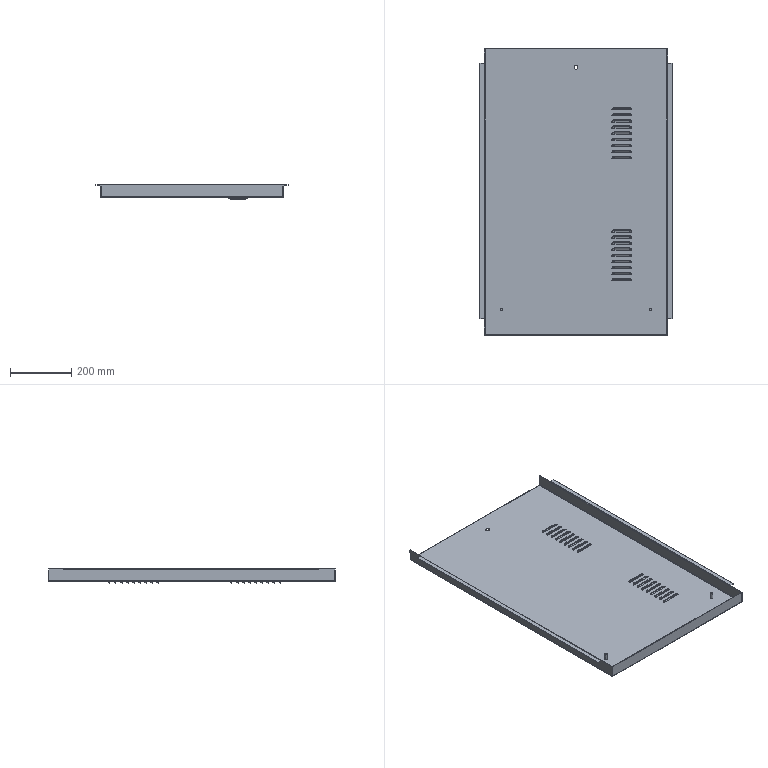Component | SolidWorks | LeftSidePlate400AType40001100-3 | 1 solid | 321 faces | volume 1026198 mm3 | plane 89 | cylinder 88 | torus 72 | sphere 72 | commonest cylinder face diameters 4 x18 12 x18 1 x18 15 x18 4.473 x5 1.473 x5 8 x4 13 x2